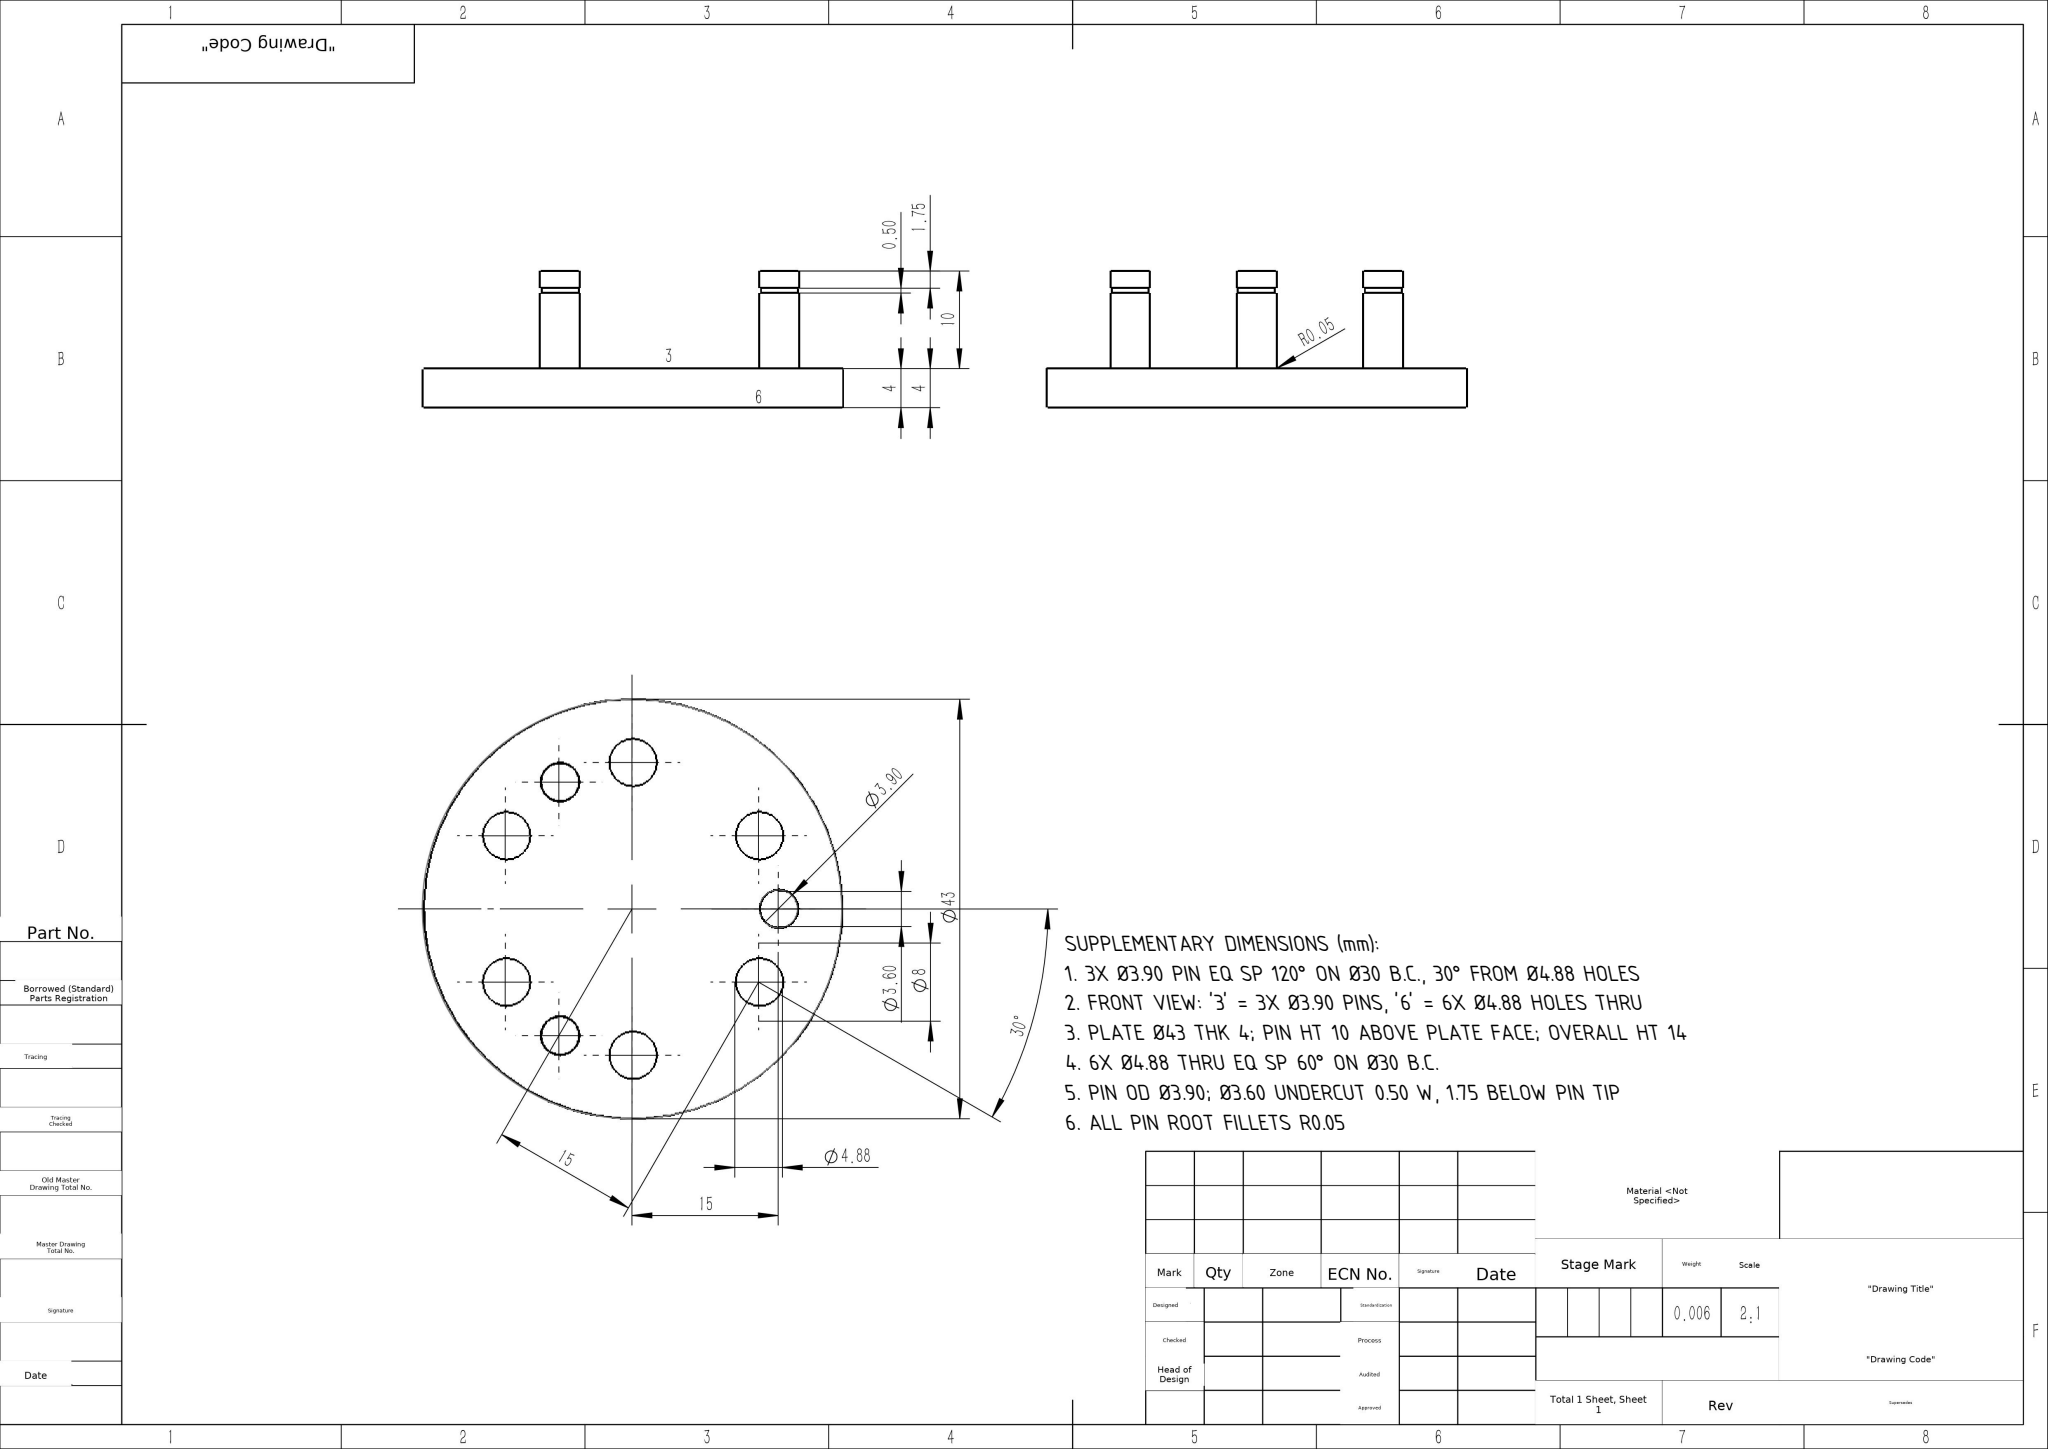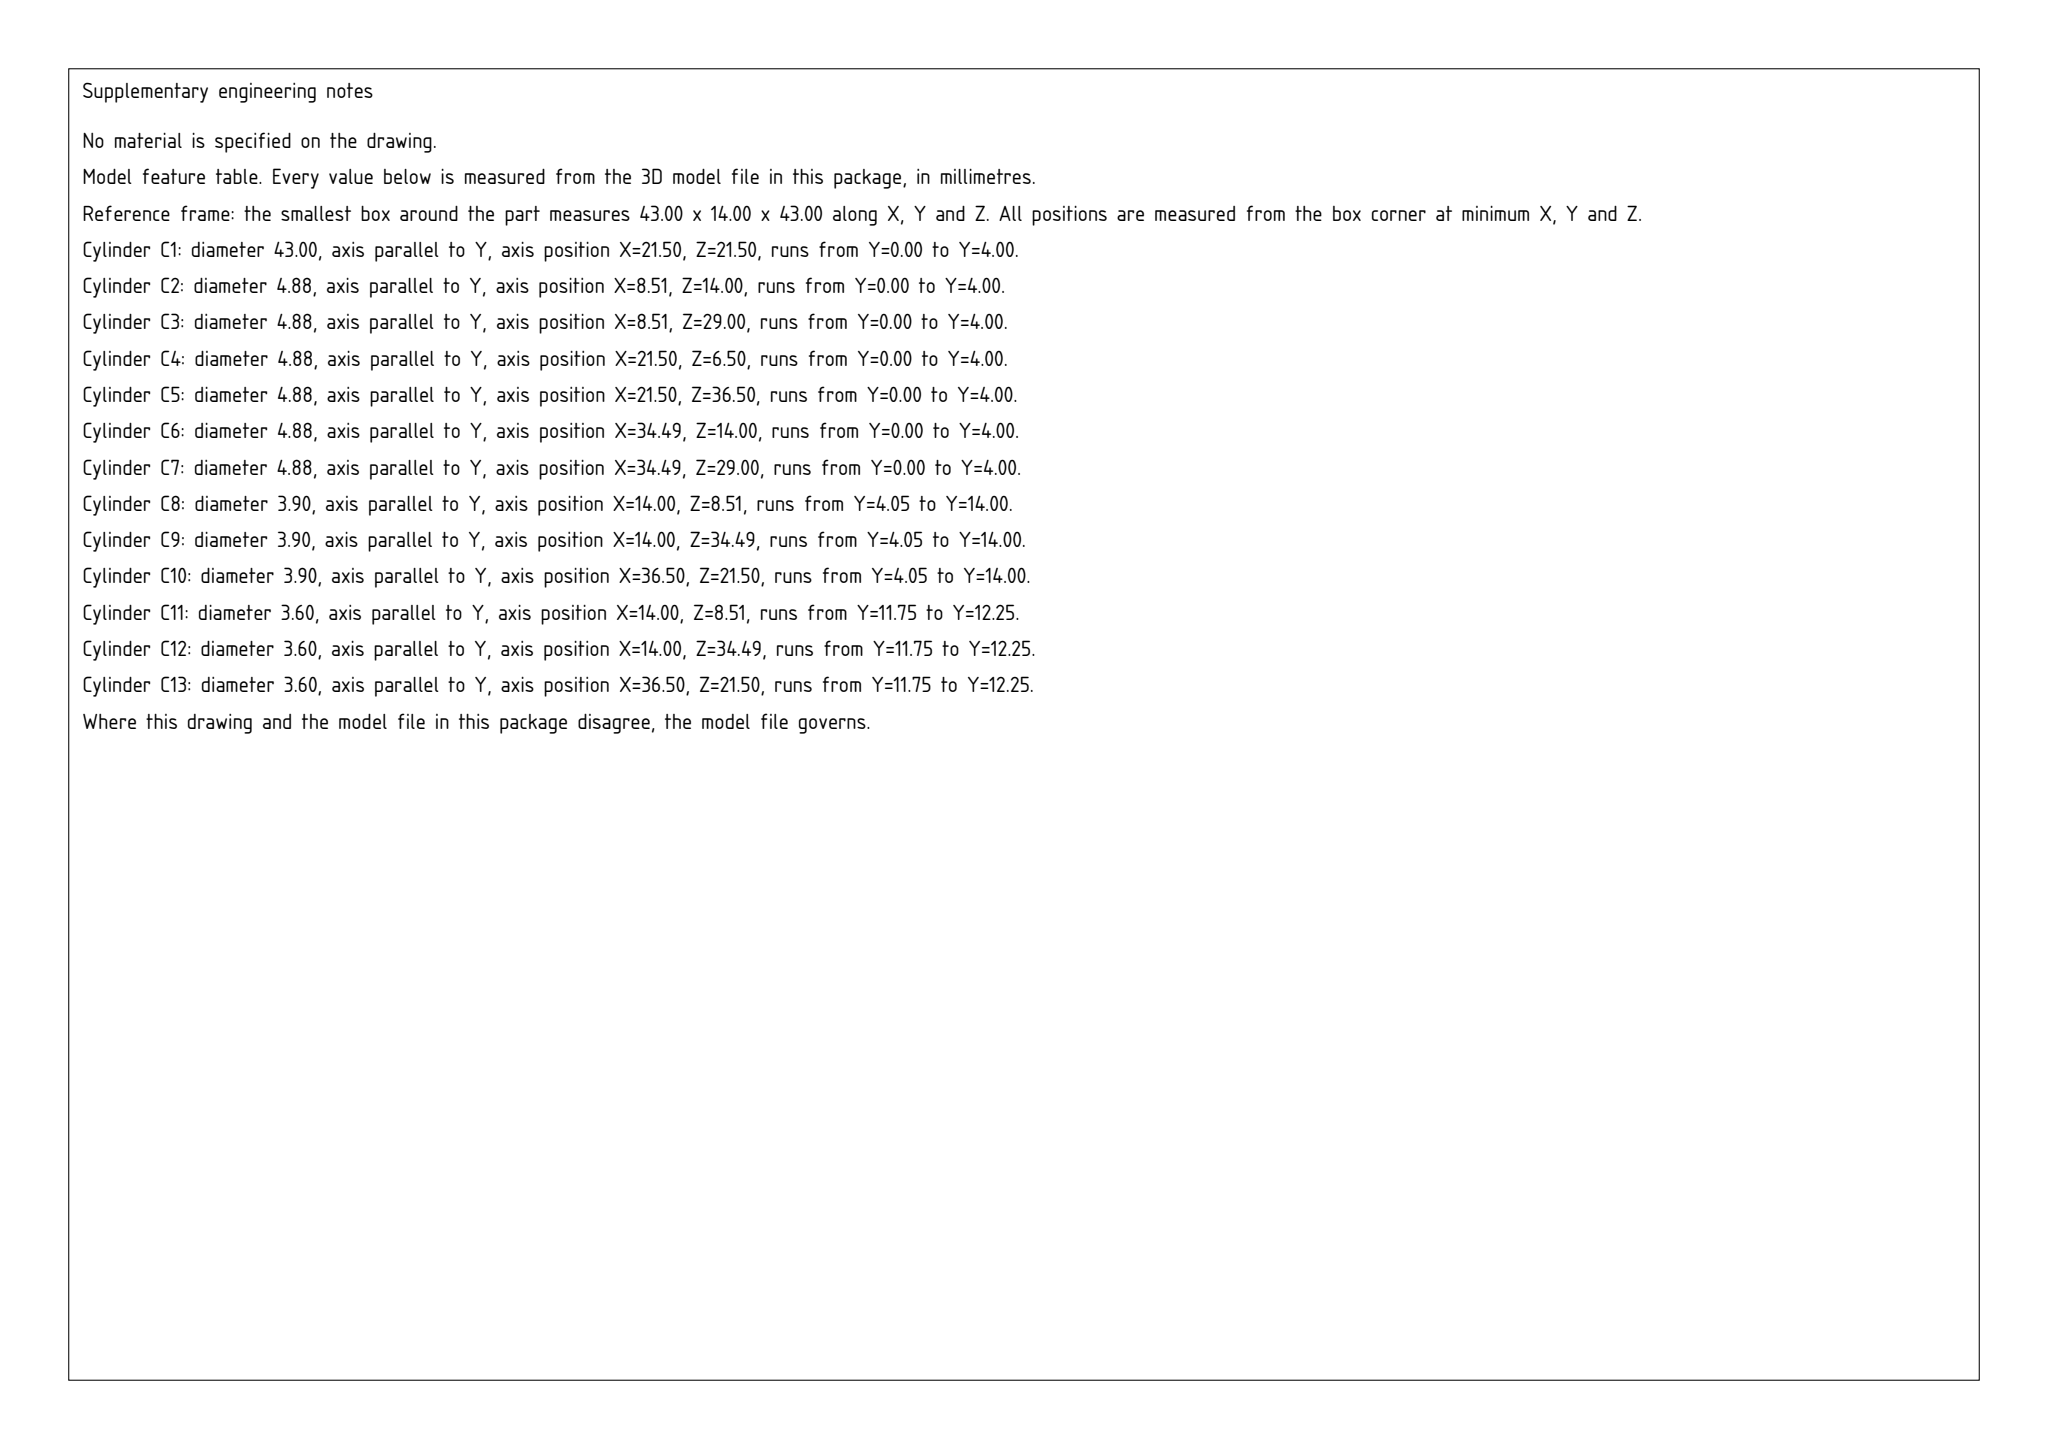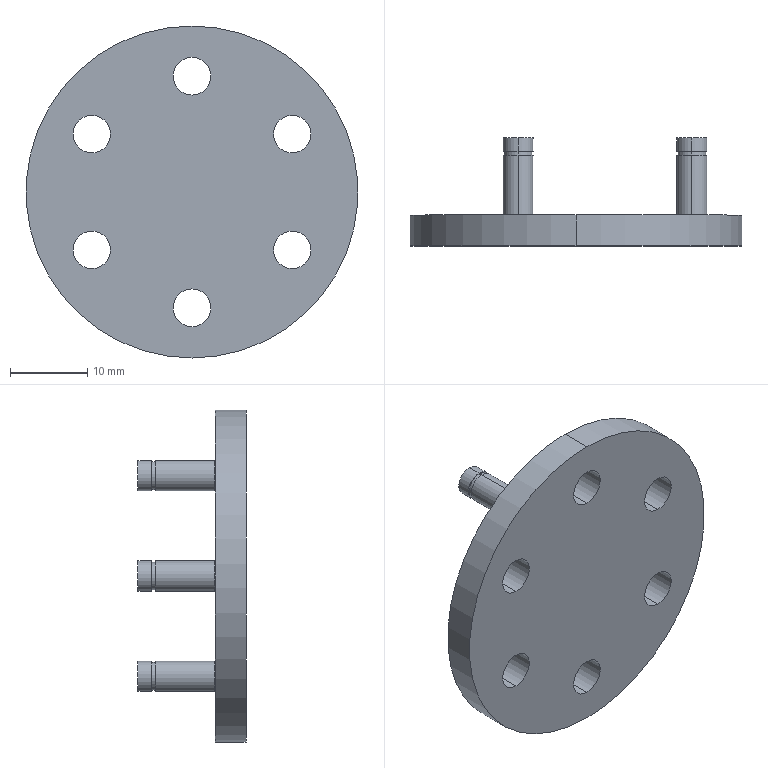Part | SolidWorks | mm | 1 solid | 49 faces | box 43 x 14 x 43 mm | volume 5716 mm3 | cylinder 32 | plane 11 | torus 6 | commonest cylinder face diameters 3.9 x12 4.88 x12 3.6 x6 43 x2
build123d program:
from build123d import *

# Parameters (mm, degrees)
SKETCH1_R           = 21.5
BOSS_EXTRUDE1_DEPTH = 4
SKETCH2_R           = 1.95
BOSS_EXTRUDE2_DEPTH = 10
FILLET1_R           = 0.05
SKETCH3_R           = 2.44
CUT_EXTRUDE1_DEPTH  = 4
CUT_EXTRUDE2_START  = -2.25
SKETCH4_R           = 1.95
SKETCH4_R_2         = 1.8
CUT_EXTRUDE2_DEPTH  = 0.5


with BuildPart() as part:
    # Sketch1 → Boss-Extrude1 (new body)
    with BuildSketch(Plane(origin=(0, 0, 0), x_dir=(1, 0, 0), z_dir=(0, 1, 0))):
        with Locations(Location((0, 0, 0), (0, 0, 270))):
            Circle(SKETCH1_R)
    extrude(amount=BOSS_EXTRUDE1_DEPTH)

    # Sketch2 → Boss-Extrude2 (add)
    with BuildSketch(Plane(origin=(0, 4, 0), x_dir=(1, 0, 0), z_dir=(0, 1, 0))):
        with Locations(Location((15, 0, 0), (0, 0, 270))):
            Circle(SKETCH2_R)
        with Locations(Location((-7.5, -12.99, 0), (0, 0, 270))):
            Circle(SKETCH2_R)
        with Locations(Location((-7.5, 12.99, 0), (0, 0, 270))):
            Circle(SKETCH2_R)
    extrude(amount=BOSS_EXTRUDE2_DEPTH)

    # Fillet1
    fillet1_edges = [part.edges().sort_by_distance(p)[0] for p in [
        (-7.5, 4, -14.94),
        (15, 4, -1.95),
        (-7.5, 4, 11.04),
    ]]
    fillet(fillet1_edges, radius=FILLET1_R)

    # Sketch3 → Cut-Extrude1 (cut)
    with BuildSketch(Plane.XZ):
        with Locations(Location((12.99, 7.5, 0), (0, 0, 270))):
            Circle(SKETCH3_R)
        with Locations(Location((12.99, -7.5, 0), (0, 0, 270))):
            Circle(SKETCH3_R)
        with Locations(Location((0, -15, 0), (0, 0, 270))):
            Circle(SKETCH3_R)
        with Locations(Location((-12.99, -7.5, 0), (0, 0, 270))):
            Circle(SKETCH3_R)
        with Locations(Location((-12.99, 7.5, 0), (0, 0, 270))):
            Circle(SKETCH3_R)
        with Locations(Location((0, 15, 0), (0, 0, 270))):
            Circle(SKETCH3_R)
    extrude(amount=-CUT_EXTRUDE1_DEPTH, mode=Mode.SUBTRACT)

    # Sketch4 → Cut-Extrude2 (cut)
    # profile 1 of 3: a face of its own
    with BuildSketch(Plane(origin=(0, 14, 0), x_dir=(1, 0, 0), z_dir=(0, 1, 0)).offset(CUT_EXTRUDE2_START)):
        with Locations(Location((-7.5, 12.99, 0), (0, 0, 270))):
            Circle(SKETCH4_R)
        with Locations(Location((-7.5, 12.99, 0), (0, 0, 270))):
            Circle(SKETCH4_R_2, mode=Mode.SUBTRACT)
    # profile 2 of 3: a face of its own
    with BuildSketch(Plane(origin=(0, 14, 0), x_dir=(1, 0, 0), z_dir=(0, 1, 0)).offset(CUT_EXTRUDE2_START)):
        with Locations(Location((15, 0, 0), (0, 0, 270))):
            Circle(SKETCH4_R)
        with Locations(Location((15, 0, 0), (0, 0, 270))):
            Circle(SKETCH4_R_2, mode=Mode.SUBTRACT)
    # profile 3 of 3: a face of its own
    with BuildSketch(Plane(origin=(0, 14, 0), x_dir=(1, 0, 0), z_dir=(0, 1, 0)).offset(CUT_EXTRUDE2_START)):
        with Locations(Location((-7.5, -12.99, 0), (0, 0, 270))):
            Circle(SKETCH4_R)
        with Locations(Location((-7.5, -12.99, 0), (0, 0, 270))):
            Circle(SKETCH4_R_2, mode=Mode.SUBTRACT)
    extrude(amount=CUT_EXTRUDE2_DEPTH, mode=Mode.SUBTRACT)


solid = part.part